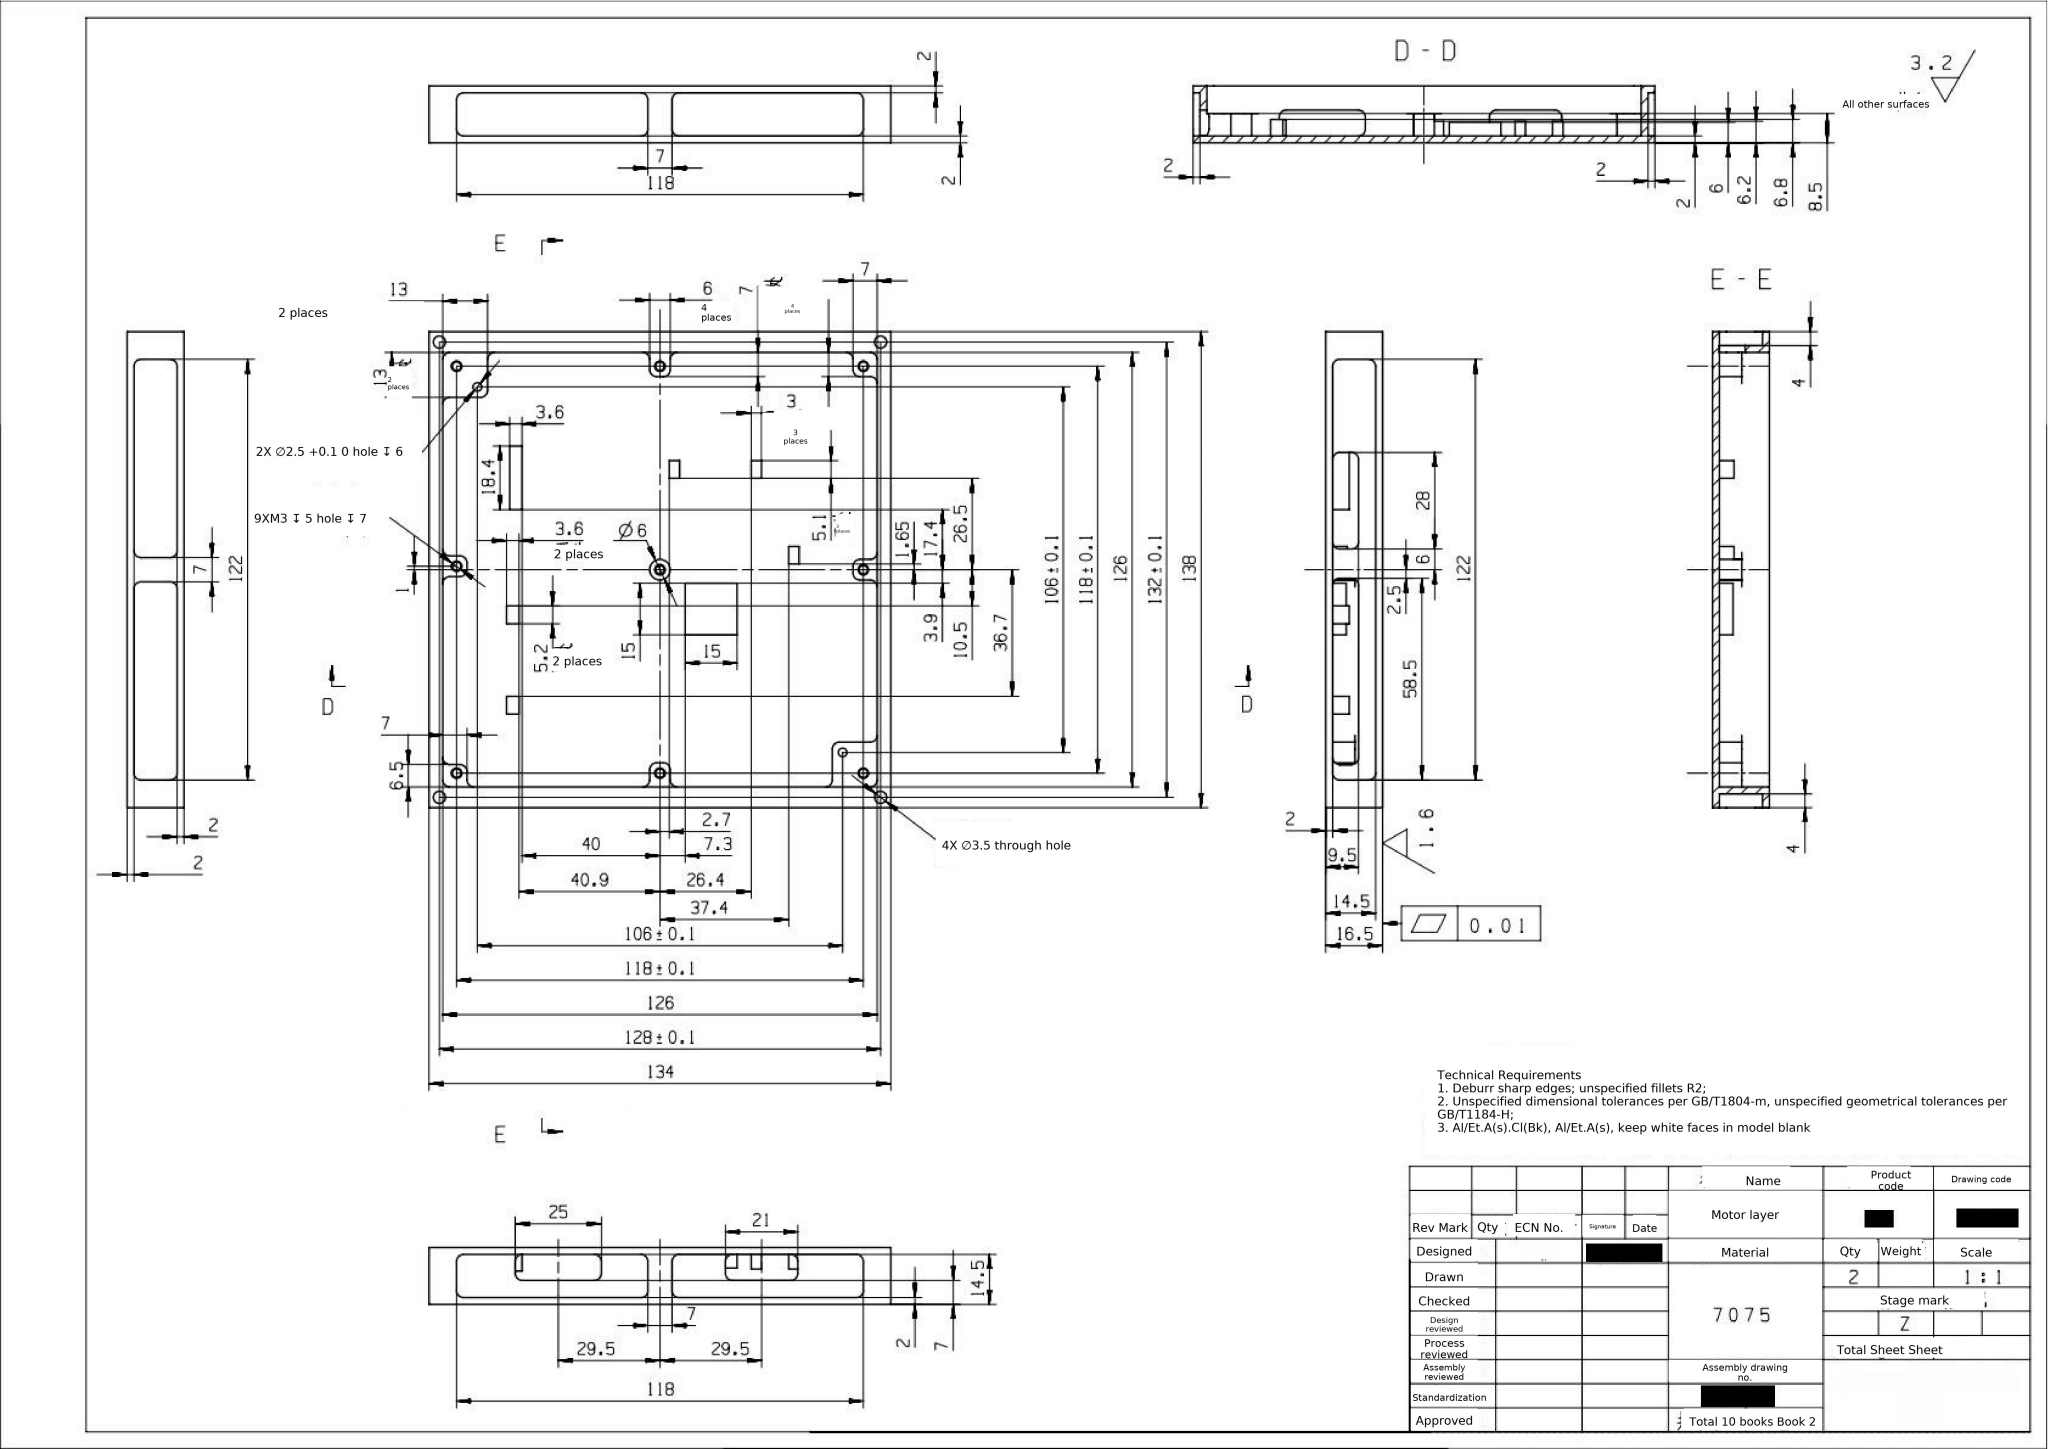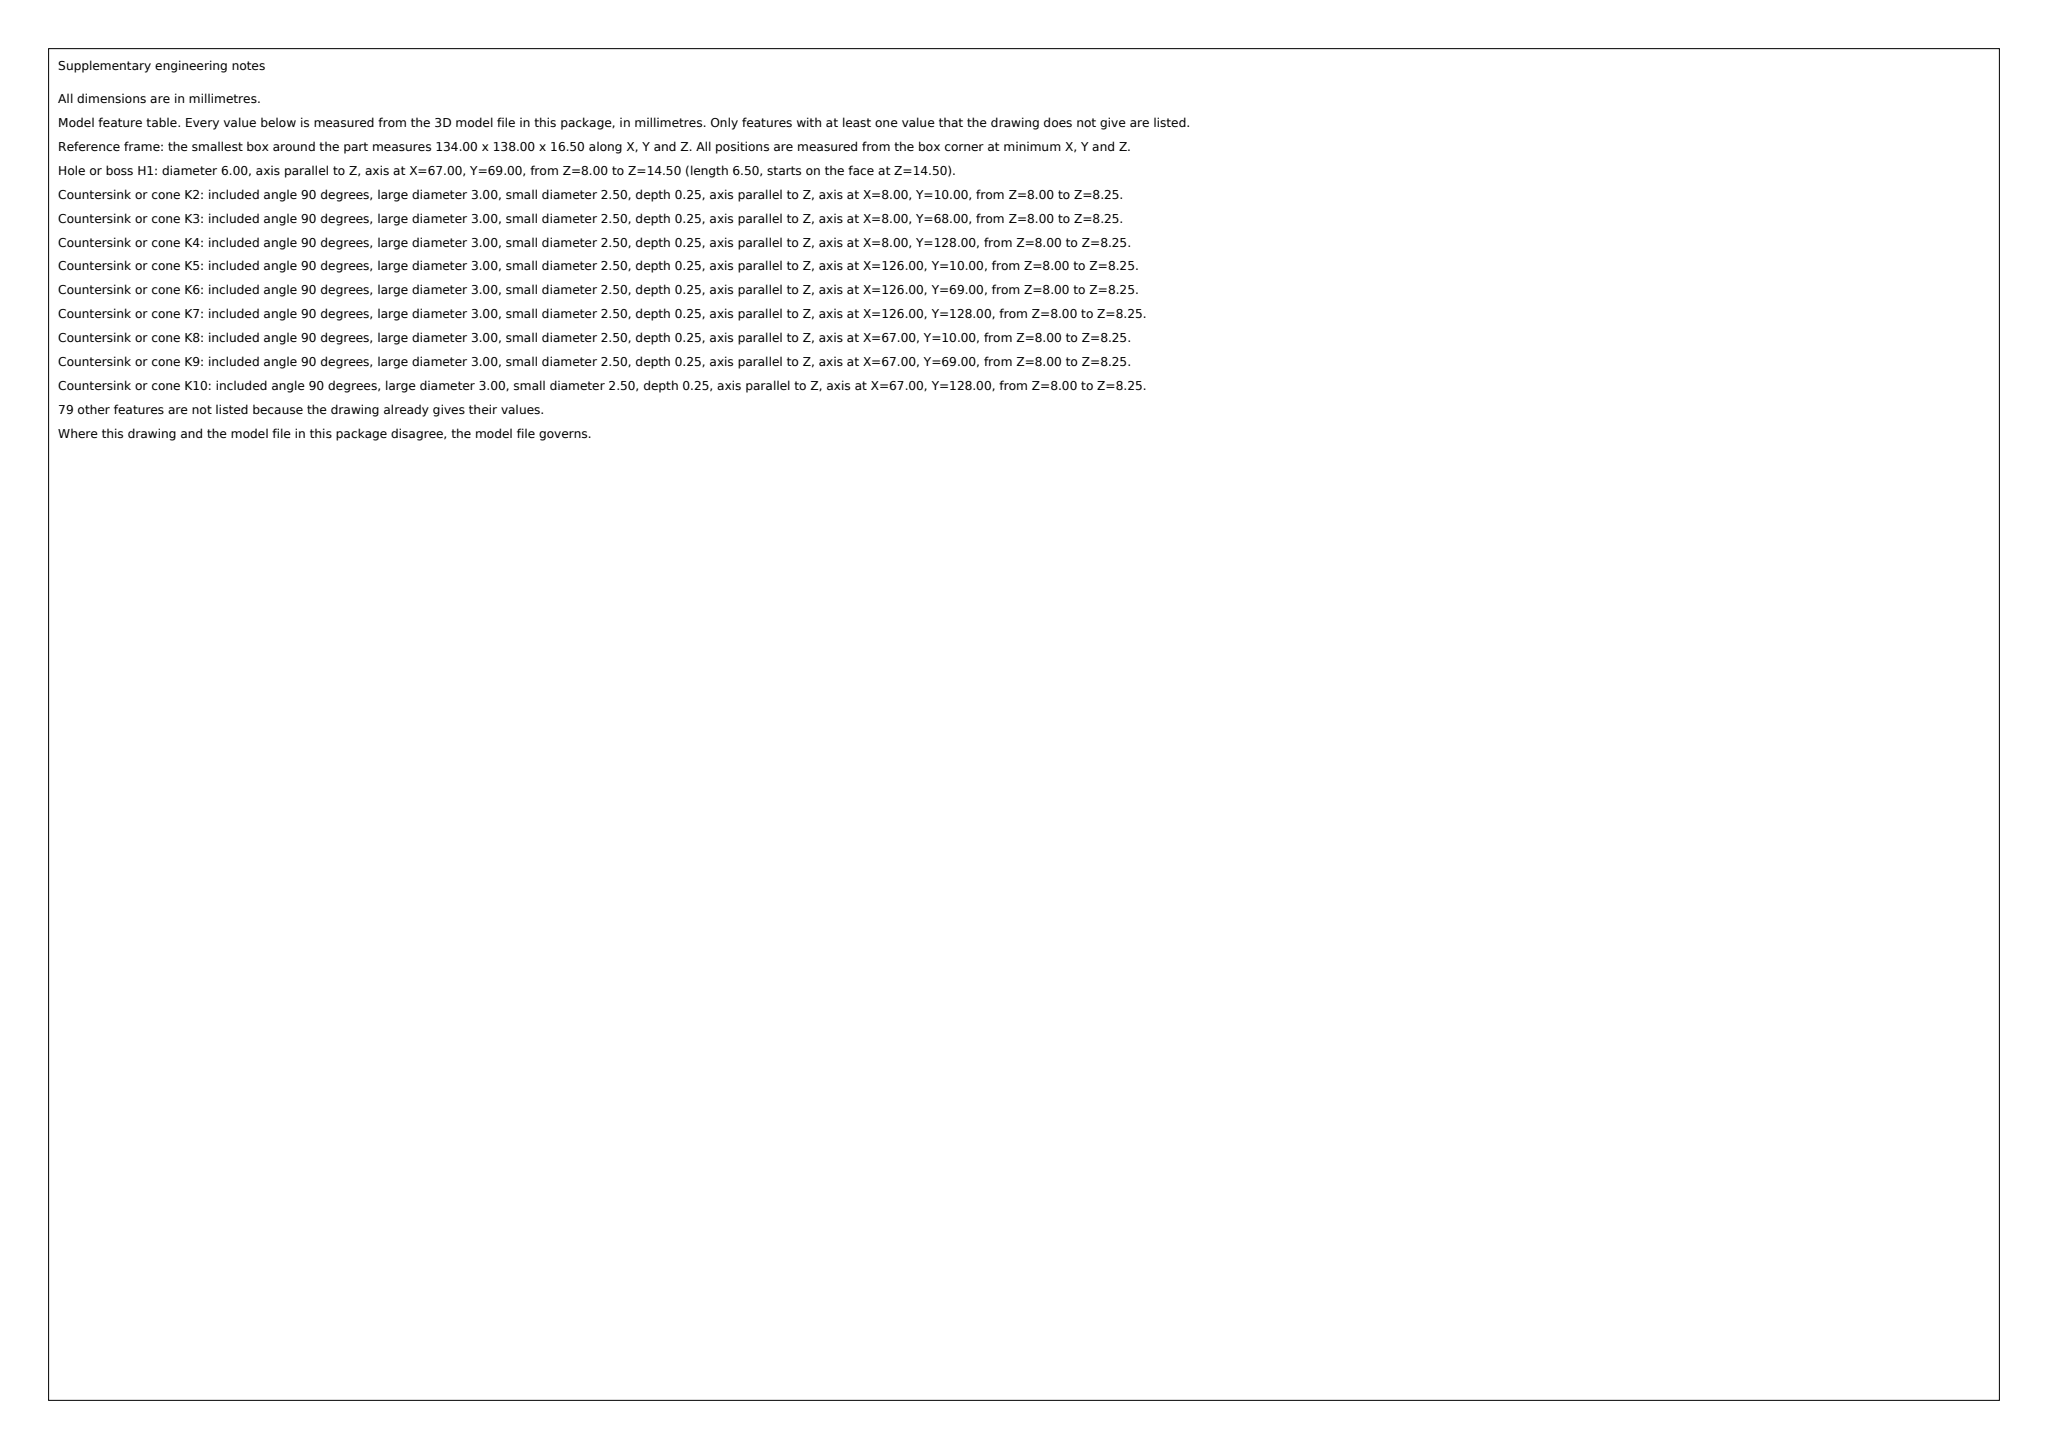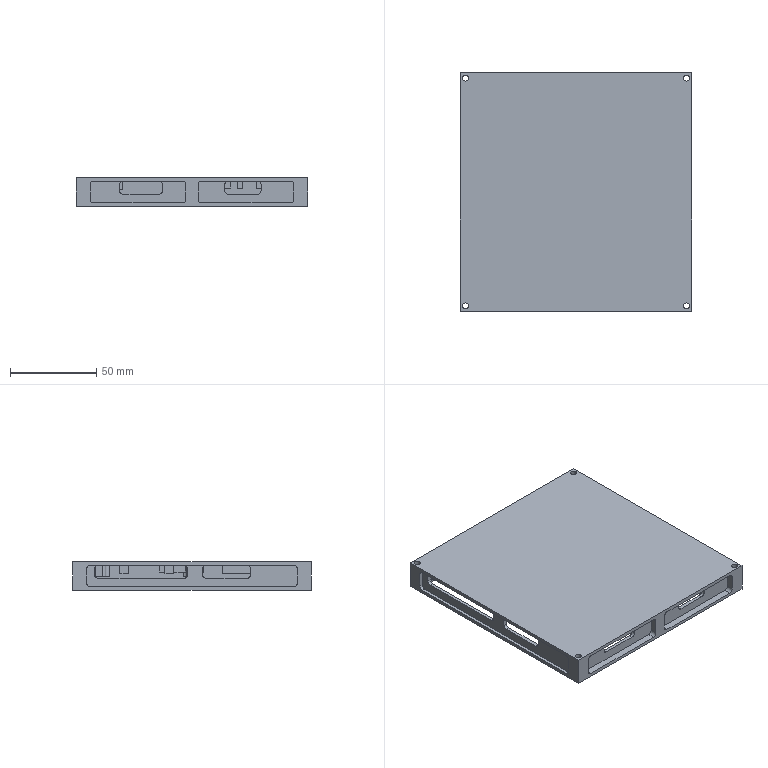Part | SolidWorks | mm | material 7075 | 1 solid | 296 faces | box 134 x 138 x 16.5 mm | volume 60765 mm3 | plane 147 | cylinder 109 | cone 40 | commonest cylinder face diameters 4 x77 2.5 x22 3.5 x8 6 x2